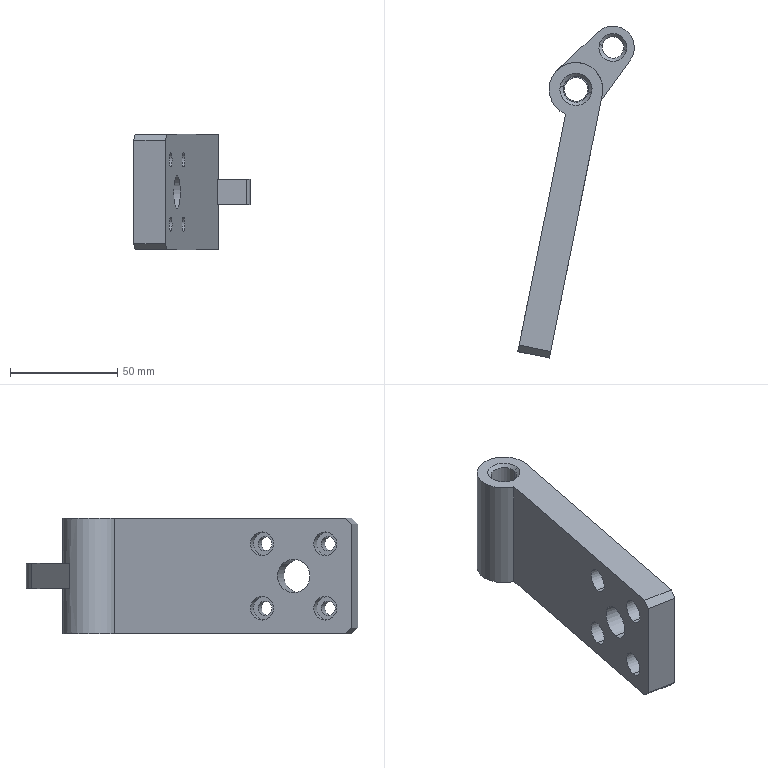Component | SolidWorks | ZTDJ-L-400-04-22-MaterialPortBagClamp-BagClampingArm-2 | 1 solid | 53 faces | box 54.27 x 154.52 x 54 mm | volume 111982 mm3 | cylinder 28 | plane 17 | cone 8 | commonest cylinder face diameters 11 x10 6.6 x8 12 x4 15.5 x2 10 x2 25 x1 20 x1 | material 1023 Carbon Steel Sheet (SS)
build123d program:
from build123d import *

# Parameters (mm, degrees)
SKETCH2_R                                            = 12.5
BOSS_EXTRUDE2_DEPTH                                  = 27
BOSS_EXTRUDE3_DEPTH                                  = 54
SKETCH5_R                                            = 5
BOSS_EXTRUDE4_DEPTH                                  = 6
SKETCH6_R                                            = 5.5
CUT_EXTRUDE1_DEPTH                                   = 139.094
SKETCH7_R                                            = 6
CUT_EXTRUDE3_DEPTH                                   = 15
CHAMFER1_SIZE                                        = 1.5
CHAMFER2_SIZE                                        = 3
HOLE_SIZE_ACCORDING_TO_THE_TYPE_OF_HEXAG_D           = 6.6
HOLE_SIZE_ACCORDING_TO_THE_TYPE_OF_HEXAG_CBORE_D     = 11
HOLE_SIZE_ACCORDING_TO_THE_TYPE_OF_HEXAG_CBORE_DEPTH = 6.8
M18_TAPPED_HOLE1_D                                   = 15.5
M18_TAPPED_HOLE1_DEPTH                               = 48.5
M18_TAPPED_HOLE1_TIP                                 = 4.657


with BuildPart() as part:
    # Sketch2 → Boss-Extrude2 (new, symmetric)
    with BuildSketch(Plane.XY):
        Circle(SKETCH2_R)
    extrude(amount=BOSS_EXTRUDE2_DEPTH, both=True)

    # Sketch3 → Boss-Extrude3 (add)
    with BuildSketch(Plane.XY.offset(27)):
        with BuildLine():
            Line((-12.5, -15), (-12.5, 0))
            ThreePointArc((-12.5, 0), (-7.906, -9.682), (2.5, -12.247))
            Line((2.5, -12.247), (2.5, -125))
            Line((2.5, -125), (-12.5, -125))
            Line((-12.5, -125), (-12.5, -15))
        make_face()
    extrude(amount=-BOSS_EXTRUDE3_DEPTH)

    # Sketch5 → Boss-Extrude4 (add, symmetric)
    with BuildSketch(Plane.XY):
        with BuildLine():
            Line((-22.101, 18.373), (-11.376, -5.18))
            ThreePointArc((-11.376, -5.18), (-6.25, 10.825), (10.174, 7.262))
            Line((10.174, 7.262), (-4.861, 28.326))
            ThreePointArc((-4.861, 28.326), (-18, 31.177), (-22.101, 18.373))
        make_face()
        with Locations((-13, 22.517)):
            Circle(SKETCH5_R, mode=Mode.SUBTRACT)
    extrude(amount=BOSS_EXTRUDE4_DEPTH, both=True)

    # Sketch6 → Cut-Extrude1 (cut, through all)
    with BuildSketch(Plane.XY.offset(27)):
        Circle(SKETCH6_R)
    extrude(amount=-CUT_EXTRUDE1_DEPTH, mode=Mode.SUBTRACT)

    # Sketch7 → Cut-Extrude3 (cut)
    with BuildSketch(Plane.XY.offset(27)):
        Circle(SKETCH7_R)
    cut_extrude3 = extrude(amount=-CUT_EXTRUDE3_DEPTH, mode=Mode.SUBTRACT)

    # Mirror2: Cut-Extrude3 across plane
    add(cut_extrude3.mirror(Plane.XY), mode=Mode.SUBTRACT)

    # Chamfer1
    chamfer1_edges = [part.edges().sort_by_distance(p)[0] for p in [
        (-18, 22.517, -6),
        (-18, 22.517, 6),
        (-6, 0, 27),
        (-6, 0, -27),
    ]]
    chamfer(chamfer1_edges, length=CHAMFER1_SIZE)

    # Chamfer2
    chamfer2_edges = [part.edges().sort_by_distance(p)[0] for p in [
        (-5, -125, 27),
        (-5, -125, -27),
    ]]
    chamfer(chamfer2_edges, length=CHAMFER2_SIZE)

    # Hole Size according to the type of Hexag (through all)
    with Locations(Plane(origin=(2.5, 0, 0), x_dir=(0, 0, -1), z_dir=(1, 0, 0))):
        with Locations((-15, -82.5), (-15, -112.5), (15, -112.5), (15, -82.5)):
            CounterBoreHole(HOLE_SIZE_ACCORDING_TO_THE_TYPE_OF_HEXAG_D / 2, HOLE_SIZE_ACCORDING_TO_THE_TYPE_OF_HEXAG_CBORE_D / 2, HOLE_SIZE_ACCORDING_TO_THE_TYPE_OF_HEXAG_CBORE_DEPTH)

    # M18 Tapped Hole1
    with Locations(Plane(origin=(2.5, 0, 0), x_dir=(0, 0, -1), z_dir=(1, 0, 0))):
        with Locations((0, -97.5)):
            Hole(M18_TAPPED_HOLE1_D / 2, depth=M18_TAPPED_HOLE1_DEPTH)
            with Locations((0, 0, -(M18_TAPPED_HOLE1_DEPTH + M18_TAPPED_HOLE1_TIP / 2))):  # 118° drill point
                Cone(0, M18_TAPPED_HOLE1_D / 2, M18_TAPPED_HOLE1_TIP, mode=Mode.SUBTRACT)


solid = part.part

# Placed as in the assembly
solid = solid.moved(Location((-88.439, -84.186, 290), (180, 0, -168.633)))